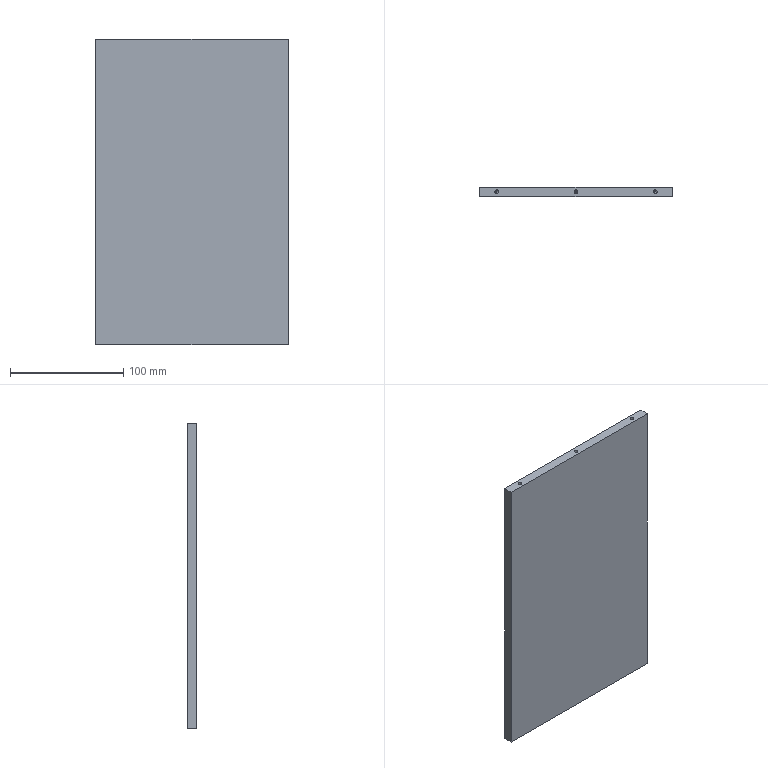Component | SolidWorks | LD101-02--Q1014-Q1-2-1 | 1 solid | 30 faces | box 170 x 8 x 270 mm | volume 366562 mm3 | cylinder 12 | cone 12 | plane 6 | commonest cylinder face diameters 3.3 x12 | material AL6061
build123d program:
from build123d import *

# Parameters (mm, degrees)
SKETCH1_W                  = 170
SKETCH1_H                  = 8
BOSS_EXTRUDE1_DEPTH        = 135
M4_TAPPED_HOLE1_AT_2_COUNT = 2
M4_TAPPED_HOLE1_AT_2_PITCH = 140
M4_TAPPED_HOLE1_AT_3_COUNT = 2
M4_TAPPED_HOLE1_AT_3_PITCH = 70


with BuildPart() as part:
    # Sketch1 → Boss-Extrude1 (new, symmetric)
    with BuildSketch(Plane.XY):
        Rectangle(SKETCH1_W, SKETCH1_H)
    extrude(amount=BOSS_EXTRUDE1_DEPTH, both=True)

    # Sketch2 → M4 Tapped Hole1 (revolve, cut)
    with BuildSketch(Plane(origin=(70, 0, -135), x_dir=(0, 1, 0), z_dir=(1, 0, 0))):
        Polygon((0, 0), (0, 13.091), (1.65, 12.1), (1.65, 0), align=None)
    m4_tapped_hole1 = revolve(axis=Axis((70, 0, -141.35), (0, 0, 1)), mode=Mode.SUBTRACT)

    # M4 Tapped Hole1 at 2: M4 Tapped Hole1 ×2
    with Locations(*[(-i * M4_TAPPED_HOLE1_AT_2_PITCH, 0, 0) for i in range(1, M4_TAPPED_HOLE1_AT_2_COUNT)]):
        add(m4_tapped_hole1, mode=Mode.SUBTRACT)

    # M4 Tapped Hole1 at 3: M4 Tapped Hole1 ×2
    with Locations(*[(-i * M4_TAPPED_HOLE1_AT_3_PITCH, 0, 0) for i in range(1, M4_TAPPED_HOLE1_AT_3_COUNT)]):
        add(m4_tapped_hole1, mode=Mode.SUBTRACT)

    # Mirror1: M4 Tapped Hole1 across plane
    add(m4_tapped_hole1.mirror(Plane.XY), mode=Mode.SUBTRACT)

    # Mirror1 copy 1 sketch → Mirror1 copy 1 (revolve, cut)
    with BuildSketch(Plane(origin=(-70, 0, 135), x_dir=(0, 1, 0), z_dir=(1, 0, 0))):
        Polygon((0, 0), (0, -13.091), (1.65, -12.1), (1.65, 0), align=None)
    revolve(axis=Axis((-70, 0, 141.35), (0, 0, 1)), mode=Mode.SUBTRACT)

    # Mirror1 copy 2 sketch → Mirror1 copy 2 (revolve, cut)
    with BuildSketch(Plane(origin=(0, 0, 135), x_dir=(0, 1, 0), z_dir=(1, 0, 0))):
        Polygon((0, 0), (0, -13.091), (1.65, -12.1), (1.65, 0), align=None)
    revolve(axis=Axis((0, 0, 141.35), (0, 0, 1)), mode=Mode.SUBTRACT)


solid = part.part

# Placed as in the assembly
solid = solid.moved(Location((244.21, -200.897, 146.257), (0, 0, 0)))
STEP:
#1=COLOUR_RGB('',0.7922,0.8196,0.9333);
#2=FILL_AREA_STYLE_COLOUR('',#1);
#3=FILL_AREA_STYLE('',(#2));
#4=SURFACE_STYLE_FILL_AREA(#3);
#5=SURFACE_SIDE_STYLE('',(#4));
#6=SURFACE_STYLE_USAGE(.BOTH.,#5);
#7=PRESENTATION_STYLE_ASSIGNMENT((#6));
#8=CARTESIAN_POINT('',(12.306,-7.909,10.597));
#9=VERTEX_POINT('',#8);
#10=CARTESIAN_POINT('',(12.435,-7.909,10.597));
#11=VERTEX_POINT('',#10);
#12=CARTESIAN_POINT('',(12.37,-7.909,10.597));
#13=DIRECTION('',(0.,0.,1.));
#14=DIRECTION('',(1.,0.,0.));
#15=AXIS2_PLACEMENT_3D('',#12,#13,#14);
#16=CIRCLE('',#15,0.06496);
#17=EDGE_CURVE('',#9,#11,#16,.T.);
#18=ORIENTED_EDGE('',*,*,#17,.F.);
#19=CARTESIAN_POINT('',(12.306,-7.909,11.073));
#20=VERTEX_POINT('',#19);
#21=CARTESIAN_POINT('',(12.306,-7.909,11.073));
#22=DIRECTION('',(0.,0.,1.));
#23=VECTOR('',#22,39.37);
#24=LINE('',#21,#23);
#25=EDGE_CURVE('',#9,#20,#24,.T.);
#26=ORIENTED_EDGE('',*,*,#25,.T.);
#27=CARTESIAN_POINT('',(12.435,-7.909,11.073));
#28=VERTEX_POINT('',#27);
#29=CARTESIAN_POINT('',(12.37,-7.909,11.073));
#30=DIRECTION('',(0.,0.,1.));
#31=DIRECTION('',(1.,0.,0.));
#32=AXIS2_PLACEMENT_3D('',#29,#30,#31);
#33=CIRCLE('',#32,0.06496);
#34=EDGE_CURVE('',#20,#28,#33,.T.);
#35=ORIENTED_EDGE('',*,*,#34,.T.);
#36=CARTESIAN_POINT('',(12.435,-7.909,11.073));
#37=DIRECTION('',(0.,0.,1.));
#38=VECTOR('',#37,39.37);
#39=LINE('',#36,#38);
#40=EDGE_CURVE('',#11,#28,#39,.T.);
#41=ORIENTED_EDGE('',*,*,#40,.F.);
#42=EDGE_LOOP('',(#18,#26,#35,#41));
#43=FACE_OUTER_BOUND('',#42,.T.);
#44=CARTESIAN_POINT('',(12.37,-7.909,11.073));
#45=DIRECTION('',(0.,0.,1.));
#46=DIRECTION('',(1.,0.,0.));
#47=AXIS2_PLACEMENT_3D('',#44,#45,#46);
#48=CYLINDRICAL_SURFACE('',#47,0.06496);
#49=ADVANCED_FACE('',(#43),#48,.F.);
#50=CARTESIAN_POINT('',(12.37,-7.909,10.558));
#51=VERTEX_POINT('',#50);
#52=CARTESIAN_POINT('',(12.435,-7.909,10.597));
#53=DIRECTION('',(0.8572,0.,0.515));
#54=VECTOR('',#53,39.37);
#55=LINE('',#52,#54);
#56=EDGE_CURVE('',#51,#11,#55,.T.);
#57=ORIENTED_EDGE('',*,*,#56,.F.);
#58=CARTESIAN_POINT('',(12.306,-7.909,10.597));
#59=DIRECTION('',(-0.8572,0.,0.515));
#60=VECTOR('',#59,39.37);
#61=LINE('',#58,#60);
#62=EDGE_CURVE('',#51,#9,#61,.T.);
#63=ORIENTED_EDGE('',*,*,#62,.T.);
#64=ORIENTED_EDGE('',*,*,#17,.T.);
#65=EDGE_LOOP('',(#57,#63,#64));
#66=FACE_OUTER_BOUND('',#65,.T.);
#67=CARTESIAN_POINT('',(12.37,-7.909,10.597));
#68=DIRECTION('',(0.,0.,1.));
#69=DIRECTION('',(1.,0.,0.));
#70=AXIS2_PLACEMENT_3D('',#67,#68,#69);
#71=CONICAL_SURFACE('',#70,0.06496,1.03);
#72=ADVANCED_FACE('',(#66),#71,.F.);
#73=CARTESIAN_POINT('',(6.794,-7.909,10.597));
#74=VERTEX_POINT('',#73);
#75=CARTESIAN_POINT('',(6.924,-7.909,10.597));
#76=VERTEX_POINT('',#75);
#77=CARTESIAN_POINT('',(6.859,-7.909,10.597));
#78=DIRECTION('',(0.,0.,1.));
#79=DIRECTION('',(1.,0.,0.));
#80=AXIS2_PLACEMENT_3D('',#77,#78,#79);
#81=CIRCLE('',#80,0.06496);
#82=EDGE_CURVE('',#74,#76,#81,.T.);
#83=ORIENTED_EDGE('',*,*,#82,.F.);
#84=CARTESIAN_POINT('',(6.794,-7.909,11.073));
#85=VERTEX_POINT('',#84);
#86=CARTESIAN_POINT('',(6.794,-7.909,11.073));
#87=DIRECTION('',(0.,0.,1.));
#88=VECTOR('',#87,39.37);
#89=LINE('',#86,#88);
#90=EDGE_CURVE('',#74,#85,#89,.T.);
#91=ORIENTED_EDGE('',*,*,#90,.T.);
#92=CARTESIAN_POINT('',(6.924,-7.909,11.073));
#93=VERTEX_POINT('',#92);
#94=CARTESIAN_POINT('',(6.859,-7.909,11.073));
#95=DIRECTION('',(0.,0.,1.));
#96=DIRECTION('',(1.,0.,0.));
#97=AXIS2_PLACEMENT_3D('',#94,#95,#96);
#98=CIRCLE('',#97,0.06496);
#99=EDGE_CURVE('',#85,#93,#98,.T.);
#100=ORIENTED_EDGE('',*,*,#99,.T.);
#101=CARTESIAN_POINT('',(6.924,-7.909,11.073));
#102=DIRECTION('',(0.,0.,1.));
#103=VECTOR('',#102,39.37);
#104=LINE('',#101,#103);
#105=EDGE_CURVE('',#76,#93,#104,.T.);
#106=ORIENTED_EDGE('',*,*,#105,.F.);
#107=EDGE_LOOP('',(#83,#91,#100,#106));
#108=FACE_OUTER_BOUND('',#107,.T.);
#109=CARTESIAN_POINT('',(6.859,-7.909,11.073));
#110=DIRECTION('',(0.,0.,1.));
#111=DIRECTION('',(1.,0.,0.));
#112=AXIS2_PLACEMENT_3D('',#109,#110,#111);
#113=CYLINDRICAL_SURFACE('',#112,0.06496);
#114=ADVANCED_FACE('',(#108),#113,.F.);
#115=CARTESIAN_POINT('',(6.859,-7.909,10.558));
#116=VERTEX_POINT('',#115);
#117=CARTESIAN_POINT('',(6.924,-7.909,10.597));
#118=DIRECTION('',(0.8572,0.,0.515));
#119=VECTOR('',#118,39.37);
#120=LINE('',#117,#119);
#121=EDGE_CURVE('',#116,#76,#120,.T.);
#122=ORIENTED_EDGE('',*,*,#121,.F.);
#123=CARTESIAN_POINT('',(6.794,-7.909,10.597));
#124=DIRECTION('',(-0.8572,0.,0.515));
#125=VECTOR('',#124,39.37);
#126=LINE('',#123,#125);
#127=EDGE_CURVE('',#116,#74,#126,.T.);
#128=ORIENTED_EDGE('',*,*,#127,.T.);
#129=ORIENTED_EDGE('',*,*,#82,.T.);
#130=EDGE_LOOP('',(#122,#128,#129));
#131=FACE_OUTER_BOUND('',#130,.T.);
#132=CARTESIAN_POINT('',(6.859,-7.909,10.597));
#133=DIRECTION('',(0.,0.,1.));
#134=DIRECTION('',(1.,0.,0.));
#135=AXIS2_PLACEMENT_3D('',#132,#133,#134);
#136=CONICAL_SURFACE('',#135,0.06496,1.03);
#137=ADVANCED_FACE('',(#131),#136,.F.);
#138=CARTESIAN_POINT('',(9.55,-7.909,10.597));
#139=VERTEX_POINT('',#138);
#140=CARTESIAN_POINT('',(9.68,-7.909,10.597));
#141=VERTEX_POINT('',#140);
#142=CARTESIAN_POINT('',(9.615,-7.909,10.597));
#143=DIRECTION('',(0.,0.,1.));
#144=DIRECTION('',(1.,0.,0.));
#145=AXIS2_PLACEMENT_3D('',#142,#143,#144);
#146=CIRCLE('',#145,0.06496);
#147=EDGE_CURVE('',#139,#141,#146,.T.);
#148=ORIENTED_EDGE('',*,*,#147,.F.);
#149=CARTESIAN_POINT('',(9.55,-7.909,11.073));
#150=VERTEX_POINT('',#149);
#151=CARTESIAN_POINT('',(9.55,-7.909,11.073));
#152=DIRECTION('',(0.,0.,1.));
#153=VECTOR('',#152,39.37);
#154=LINE('',#151,#153);
#155=EDGE_CURVE('',#139,#150,#154,.T.);
#156=ORIENTED_EDGE('',*,*,#155,.T.);
#157=CARTESIAN_POINT('',(9.68,-7.909,11.073));
#158=VERTEX_POINT('',#157);
#159=CARTESIAN_POINT('',(9.615,-7.909,11.073));
#160=DIRECTION('',(0.,0.,1.));
#161=DIRECTION('',(1.,0.,0.));
#162=AXIS2_PLACEMENT_3D('',#159,#160,#161);
#163=CIRCLE('',#162,0.06496);
#164=EDGE_CURVE('',#150,#158,#163,.T.);
#165=ORIENTED_EDGE('',*,*,#164,.T.);
#166=CARTESIAN_POINT('',(9.68,-7.909,11.073));
#167=DIRECTION('',(0.,0.,1.));
#168=VECTOR('',#167,39.37);
#169=LINE('',#166,#168);
#170=EDGE_CURVE('',#141,#158,#169,.T.);
#171=ORIENTED_EDGE('',*,*,#170,.F.);
#172=EDGE_LOOP('',(#148,#156,#165,#171));
#173=FACE_OUTER_BOUND('',#172,.T.);
#174=CARTESIAN_POINT('',(9.615,-7.909,11.073));
#175=DIRECTION('',(0.,0.,1.));
#176=DIRECTION('',(1.,0.,0.));
#177=AXIS2_PLACEMENT_3D('',#174,#175,#176);
#178=CYLINDRICAL_SURFACE('',#177,0.06496);
#179=ADVANCED_FACE('',(#173),#178,.F.);
#180=CARTESIAN_POINT('',(9.615,-7.909,10.558));
#181=VERTEX_POINT('',#180);
#182=CARTESIAN_POINT('',(9.68,-7.909,10.597));
#183=DIRECTION('',(0.8572,0.,0.515));
#184=VECTOR('',#183,39.37);
#185=LINE('',#182,#184);
#186=EDGE_CURVE('',#181,#141,#185,.T.);
#187=ORIENTED_EDGE('',*,*,#186,.F.);
#188=CARTESIAN_POINT('',(9.55,-7.909,10.597));
#189=DIRECTION('',(-0.8572,0.,0.515));
#190=VECTOR('',#189,39.37);
#191=LINE('',#188,#190);
#192=EDGE_CURVE('',#181,#139,#191,.T.);
#193=ORIENTED_EDGE('',*,*,#192,.T.);
#194=ORIENTED_EDGE('',*,*,#147,.T.);
#195=EDGE_LOOP('',(#187,#193,#194));
#196=FACE_OUTER_BOUND('',#195,.T.);
#197=CARTESIAN_POINT('',(9.615,-7.909,10.597));
#198=DIRECTION('',(0.,0.,1.));
#199=DIRECTION('',(1.,0.,0.));
#200=AXIS2_PLACEMENT_3D('',#197,#198,#199);
#201=CONICAL_SURFACE('',#200,0.06496,1.03);
#202=ADVANCED_FACE('',(#196),#201,.F.);
#203=CARTESIAN_POINT('',(12.435,-7.909,0.9196));
#204=VERTEX_POINT('',#203);
#205=CARTESIAN_POINT('',(12.306,-7.909,0.9196));
#206=VERTEX_POINT('',#205);
#207=CARTESIAN_POINT('',(12.37,-7.909,0.9196));
#208=DIRECTION('',(0.,0.,-1.));
#209=DIRECTION('',(-1.,0.,0.));
#210=AXIS2_PLACEMENT_3D('',#207,#208,#209);
#211=CIRCLE('',#210,0.06496);
#212=EDGE_CURVE('',#204,#206,#211,.T.);
#213=ORIENTED_EDGE('',*,*,#212,.F.);
#214=CARTESIAN_POINT('',(12.435,-7.909,0.4432));
#215=VERTEX_POINT('',#214);
#216=CARTESIAN_POINT('',(12.435,-7.909,0.4432));
#217=DIRECTION('',(0.,0.,-1.));
#218=VECTOR('',#217,39.37);
#219=LINE('',#216,#218);
#220=EDGE_CURVE('',#204,#215,#219,.T.);
#221=ORIENTED_EDGE('',*,*,#220,.T.);
#222=CARTESIAN_POINT('',(12.306,-7.909,0.4432));
#223=VERTEX_POINT('',#222);
#224=CARTESIAN_POINT('',(12.37,-7.909,0.4432));
#225=DIRECTION('',(0.,0.,-1.));
#226=DIRECTION('',(-1.,0.,0.));
#227=AXIS2_PLACEMENT_3D('',#224,#225,#226);
#228=CIRCLE('',#227,0.06496);
#229=EDGE_CURVE('',#215,#223,#228,.T.);
#230=ORIENTED_EDGE('',*,*,#229,.T.);
#231=CARTESIAN_POINT('',(12.306,-7.909,0.4432));
#232=DIRECTION('',(0.,0.,-1.));
#233=VECTOR('',#232,39.37);
#234=LINE('',#231,#233);
#235=EDGE_CURVE('',#206,#223,#234,.T.);
#236=ORIENTED_EDGE('',*,*,#235,.F.);
#237=EDGE_LOOP('',(#213,#221,#230,#236));
#238=FACE_OUTER_BOUND('',#237,.T.);
#239=CARTESIAN_POINT('',(12.37,-7.909,0.4432));
#240=DIRECTION('',(0.,0.,-1.));
#241=DIRECTION('',(-1.,0.,0.));
#242=AXIS2_PLACEMENT_3D('',#239,#240,#241);
#243=CYLINDRICAL_SURFACE('',#242,0.06496);
#244=ADVANCED_FACE('',(#238),#243,.F.);
#245=CARTESIAN_POINT('',(12.37,-7.909,0.9586));
#246=VERTEX_POINT('',#245);
#247=CARTESIAN_POINT('',(12.306,-7.909,0.9196));
#248=DIRECTION('',(-0.8572,0.,-0.515));
#249=VECTOR('',#248,39.37);
#250=LINE('',#247,#249);
#251=EDGE_CURVE('',#246,#206,#250,.T.);
#252=ORIENTED_EDGE('',*,*,#251,.F.);
#253=CARTESIAN_POINT('',(12.435,-7.909,0.9196));
#254=DIRECTION('',(0.8572,0.,-0.515));
#255=VECTOR('',#254,39.37);
#256=LINE('',#253,#255);
#257=EDGE_CURVE('',#246,#204,#256,.T.);
#258=ORIENTED_EDGE('',*,*,#257,.T.);
#259=ORIENTED_EDGE('',*,*,#212,.T.);
#260=EDGE_LOOP('',(#252,#258,#259));
#261=FACE_OUTER_BOUND('',#260,.T.);
#262=CARTESIAN_POINT('',(12.37,-7.909,0.9196));
#263=DIRECTION('',(0.,0.,-1.));
#264=DIRECTION('',(-1.,0.,0.));
#265=AXIS2_PLACEMENT_3D('',#262,#263,#264);
#266=CONICAL_SURFACE('',#265,0.06496,1.03);
#267=ADVANCED_FACE('',(#261),#266,.F.);
#268=CARTESIAN_POINT('',(6.924,-7.909,0.9196));
#269=VERTEX_POINT('',#268);
#270=CARTESIAN_POINT('',(6.794,-7.909,0.9196));
#271=VERTEX_POINT('',#270);
#272=CARTESIAN_POINT('',(6.859,-7.909,0.9196));
#273=DIRECTION('',(0.,0.,-1.));
#274=DIRECTION('',(-1.,0.,0.));
#275=AXIS2_PLACEMENT_3D('',#272,#273,#274);
#276=CIRCLE('',#275,0.06496);
#277=EDGE_CURVE('',#269,#271,#276,.T.);
#278=ORIENTED_EDGE('',*,*,#277,.F.);
#279=CARTESIAN_POINT('',(6.924,-7.909,0.4432));
#280=VERTEX_POINT('',#279);
#281=CARTESIAN_POINT('',(6.924,-7.909,0.4432));
#282=DIRECTION('',(0.,0.,-1.));
#283=VECTOR('',#282,39.37);
#284=LINE('',#281,#283);
#285=EDGE_CURVE('',#269,#280,#284,.T.);
#286=ORIENTED_EDGE('',*,*,#285,.T.);
#287=CARTESIAN_POINT('',(6.794,-7.909,0.4432));
#288=VERTEX_POINT('',#287);
#289=CARTESIAN_POINT('',(6.859,-7.909,0.4432));
#290=DIRECTION('',(0.,0.,-1.));
#291=DIRECTION('',(-1.,0.,0.));
#292=AXIS2_PLACEMENT_3D('',#289,#290,#291);
#293=CIRCLE('',#292,0.06496);
#294=EDGE_CURVE('',#280,#288,#293,.T.);
#295=ORIENTED_EDGE('',*,*,#294,.T.);
#296=CARTESIAN_POINT('',(6.794,-7.909,0.4432));
#297=DIRECTION('',(0.,0.,-1.));
#298=VECTOR('',#297,39.37);
#299=LINE('',#296,#298);
#300=EDGE_CURVE('',#271,#288,#299,.T.);
#301=ORIENTED_EDGE('',*,*,#300,.F.);
#302=EDGE_LOOP('',(#278,#286,#295,#301));
#303=FACE_OUTER_BOUND('',#302,.T.);
#304=CARTESIAN_POINT('',(6.859,-7.909,0.4432));
#305=DIRECTION('',(0.,0.,-1.));
#306=DIRECTION('',(-1.,0.,0.));
#307=AXIS2_PLACEMENT_3D('',#304,#305,#306);
#308=CYLINDRICAL_SURFACE('',#307,0.06496);
#309=ADVANCED_FACE('',(#303),#308,.F.);
#310=CARTESIAN_POINT('',(6.859,-7.909,0.9586));
#311=VERTEX_POINT('',#310);
#312=CARTESIAN_POINT('',(6.794,-7.909,0.9196));
#313=DIRECTION('',(-0.8572,0.,-0.515));
#314=VECTOR('',#313,39.37);
#315=LINE('',#312,#314);
#316=EDGE_CURVE('',#311,#271,#315,.T.);
#317=ORIENTED_EDGE('',*,*,#316,.F.);
#318=CARTESIAN_POINT('',(6.924,-7.909,0.9196));
#319=DIRECTION('',(0.8572,0.,-0.515));
#320=VECTOR('',#319,39.37);
#321=LINE('',#318,#320);
#322=EDGE_CURVE('',#311,#269,#321,.T.);
#323=ORIENTED_EDGE('',*,*,#322,.T.);
#324=ORIENTED_EDGE('',*,*,#277,.T.);
#325=EDGE_LOOP('',(#317,#323,#324));
#326=FACE_OUTER_BOUND('',#325,.T.);
#327=CARTESIAN_POINT('',(6.859,-7.909,0.9196));
#328=DIRECTION('',(0.,0.,-1.));
#329=DIRECTION('',(-1.,0.,0.));
#330=AXIS2_PLACEMENT_3D('',#327,#328,#329);
#331=CONICAL_SURFACE('',#330,0.06496,1.03);
#332=ADVANCED_FACE('',(#326),#331,.F.);
#333=CARTESIAN_POINT('',(9.68,-7.909,0.9196));
#334=VERTEX_POINT('',#333);
#335=CARTESIAN_POINT('',(9.55,-7.909,0.9196));
#336=VERTEX_POINT('',#335);
#337=CARTESIAN_POINT('',(9.615,-7.909,0.9196));
#338=DIRECTION('',(0.,0.,-1.));
#339=DIRECTION('',(-1.,0.,0.));
#340=AXIS2_PLACEMENT_3D('',#337,#338,#339);
#341=CIRCLE('',#340,0.06496);
#342=EDGE_CURVE('',#334,#336,#341,.T.);
#343=ORIENTED_EDGE('',*,*,#342,.F.);
#344=CARTESIAN_POINT('',(9.68,-7.909,0.4432));
#345=VERTEX_POINT('',#344);
#346=CARTESIAN_POINT('',(9.68,-7.909,0.4432));
#347=DIRECTION('',(0.,0.,-1.));
#348=VECTOR('',#347,39.37);
#349=LINE('',#346,#348);
#350=EDGE_CURVE('',#334,#345,#349,.T.);
#351=ORIENTED_EDGE('',*,*,#350,.T.);
#352=CARTESIAN_POINT('',(9.55,-7.909,0.4432));
#353=VERTEX_POINT('',#352);
#354=CARTESIAN_POINT('',(9.615,-7.909,0.4432));
#355=DIRECTION('',(0.,0.,-1.));
#356=DIRECTION('',(-1.,0.,0.));
#357=AXIS2_PLACEMENT_3D('',#354,#355,#356);
#358=CIRCLE('',#357,0.06496);
#359=EDGE_CURVE('',#345,#353,#358,.T.);
#360=ORIENTED_EDGE('',*,*,#359,.T.);
#361=CARTESIAN_POINT('',(9.55,-7.909,0.4432));
#362=DIRECTION('',(0.,0.,-1.));
#363=VECTOR('',#362,39.37);
#364=LINE('',#361,#363);
#365=EDGE_CURVE('',#336,#353,#364,.T.);
#366=ORIENTED_EDGE('',*,*,#365,.F.);
#367=EDGE_LOOP('',(#343,#351,#360,#366));
#368=FACE_OUTER_BOUND('',#367,.T.);
#369=CARTESIAN_POINT('',(9.615,-7.909,0.4432));
#370=DIRECTION('',(0.,0.,-1.));
#371=DIRECTION('',(-1.,0.,0.));
#372=AXIS2_PLACEMENT_3D('',#369,#370,#371);
#373=CYLINDRICAL_SURFACE('',#372,0.06496);
#374=ADVANCED_FACE('',(#368),#373,.F.);
#375=CARTESIAN_POINT('',(9.615,-7.909,0.9586));
#376=VERTEX_POINT('',#375);
#377=CARTESIAN_POINT('',(9.55,-7.909,0.9196));
#378=DIRECTION('',(-0.8572,0.,-0.515));
#379=VECTOR('',#378,39.37);
#380=LINE('',#377,#379);
#381=EDGE_CURVE('',#376,#336,#380,.T.);
#382=ORIENTED_EDGE('',*,*,#381,.F.);
#383=CARTESIAN_POINT('',(9.68,-7.909,0.9196));
#384=DIRECTION('',(0.8572,0.,-0.515));
#385=VECTOR('',#384,39.37);
#386=LINE('',#383,#385);
#387=EDGE_CURVE('',#376,#334,#386,.T.);
#388=ORIENTED_EDGE('',*,*,#387,.T.);
#389=ORIENTED_EDGE('',*,*,#342,.T.);
#390=EDGE_LOOP('',(#382,#388,#389));
#391=FACE_OUTER_BOUND('',#390,.T.);
#392=CARTESIAN_POINT('',(9.615,-7.909,0.9196));
#393=DIRECTION('',(0.,0.,-1.));
#394=DIRECTION('',(-1.,0.,0.));
#395=AXIS2_PLACEMENT_3D('',#392,#393,#394);
#396=CONICAL_SURFACE('',#395,0.06496,1.03);
#397=ADVANCED_FACE('',(#391),#396,.F.);
#398=CARTESIAN_POINT('',(12.961,-8.067,0.4432));
#399=VERTEX_POINT('',#398);
#400=CARTESIAN_POINT('',(12.961,-7.752,0.4432));
#401=VERTEX_POINT('',#400);
#402=CARTESIAN_POINT('',(12.961,-8.067,0.4432));
#403=DIRECTION('',(0.,1.,0.));
#404=VECTOR('',#403,39.37);
#405=LINE('',#402,#404);
#406=EDGE_CURVE('',#399,#401,#405,.T.);
#407=ORIENTED_EDGE('',*,*,#406,.T.);
#408=CARTESIAN_POINT('',(12.961,-7.752,11.073));
#409=VERTEX_POINT('',#408);
#410=CARTESIAN_POINT('',(12.961,-7.752,11.073));
#411=DIRECTION('',(0.,0.,-1.));
#412=VECTOR('',#411,39.37);
#413=LINE('',#410,#412);
#414=EDGE_CURVE('',#409,#401,#413,.T.);
#415=ORIENTED_EDGE('',*,*,#414,.F.);
#416=CARTESIAN_POINT('',(12.961,-8.067,11.073));
#417=VERTEX_POINT('',#416);
#418=CARTESIAN_POINT('',(12.961,-8.067,11.073));
#419=DIRECTION('',(0.,1.,0.));
#420=VECTOR('',#419,39.37);
#421=LINE('',#418,#420);
#422=EDGE_CURVE('',#417,#409,#421,.T.);
#423=ORIENTED_EDGE('',*,*,#422,.F.);
#424=CARTESIAN_POINT('',(12.961,-8.067,11.073));
#425=DIRECTION('',(0.,0.,-1.));
#426=VECTOR('',#425,39.37);
#427=LINE('',#424,#426);
#428=EDGE_CURVE('',#417,#399,#427,.T.);
#429=ORIENTED_EDGE('',*,*,#428,.T.);
#430=EDGE_LOOP('',(#407,#415,#423,#429));
#431=FACE_OUTER_BOUND('',#430,.T.);
#432=CARTESIAN_POINT('',(12.961,-8.067,11.073));
#433=DIRECTION('',(-1.,0.,0.));
#434=DIRECTION('',(0.,0.,1.));
#435=AXIS2_PLACEMENT_3D('',#432,#433,#434);
#436=PLANE('',#435);
#437=ADVANCED_FACE('',(#431),#436,.F.);
#438=CARTESIAN_POINT('',(6.268,-7.752,0.4432));
#439=VERTEX_POINT('',#438);
#440=CARTESIAN_POINT('',(6.268,-7.752,0.4432));
#441=DIRECTION('',(-1.,0.,0.));
#442=VECTOR('',#441,39.37);
#443=LINE('',#440,#442);
#444=EDGE_CURVE('',#401,#439,#443,.T.);
#445=ORIENTED_EDGE('',*,*,#444,.T.);
#446=CARTESIAN_POINT('',(6.268,-7.752,11.073));
#447=VERTEX_POINT('',#446);
#448=CARTESIAN_POINT('',(6.268,-7.752,11.073));
#449=DIRECTION('',(0.,0.,-1.));
#450=VECTOR('',#449,39.37);
#451=LINE('',#448,#450);
#452=EDGE_CURVE('',#447,#439,#451,.T.);
#453=ORIENTED_EDGE('',*,*,#452,.F.);
#454=CARTESIAN_POINT('',(6.268,-7.752,11.073));
#455=DIRECTION('',(-1.,0.,0.));
#456=VECTOR('',#455,39.37);
#457=LINE('',#454,#456);
#458=EDGE_CURVE('',#409,#447,#457,.T.);
#459=ORIENTED_EDGE('',*,*,#458,.F.);
#460=ORIENTED_EDGE('',*,*,#414,.T.);
#461=EDGE_LOOP('',(#445,#453,#459,#460));
#462=FACE_OUTER_BOUND('',#461,.T.);
#463=CARTESIAN_POINT('',(6.268,-7.752,11.073));
#464=DIRECTION('',(0.,-1.,0.));
#465=DIRECTION('',(0.,0.,-1.));
#466=AXIS2_PLACEMENT_3D('',#463,#464,#465);
#467=PLANE('',#466);
#468=ADVANCED_FACE('',(#462),#467,.F.);
#469=CARTESIAN_POINT('',(6.268,-8.067,0.4432));
#470=VERTEX_POINT('',#469);
#471=CARTESIAN_POINT('',(6.268,-8.067,0.4432));
#472=DIRECTION('',(0.,-1.,0.));
#473=VECTOR('',#472,39.37);
#474=LINE('',#471,#473);
#475=EDGE_CURVE('',#439,#470,#474,.T.);
#476=ORIENTED_EDGE('',*,*,#475,.T.);
#477=CARTESIAN_POINT('',(6.268,-8.067,11.073));
#478=VERTEX_POINT('',#477);
#479=CARTESIAN_POINT('',(6.268,-8.067,11.073));
#480=DIRECTION('',(0.,0.,-1.));
#481=VECTOR('',#480,39.37);
#482=LINE('',#479,#481);
#483=EDGE_CURVE('',#478,#470,#482,.T.);
#484=ORIENTED_EDGE('',*,*,#483,.F.);
#485=CARTESIAN_POINT('',(6.268,-8.067,11.073));
#486=DIRECTION('',(0.,-1.,0.));
#487=VECTOR('',#486,39.37);
#488=LINE('',#485,#487);
#489=EDGE_CURVE('',#447,#478,#488,.T.);
#490=ORIENTED_EDGE('',*,*,#489,.F.);
#491=ORIENTED_EDGE('',*,*,#452,.T.);
#492=EDGE_LOOP('',(#476,#484,#490,#491));
#493=FACE_OUTER_BOUND('',#492,.T.);
#494=CARTESIAN_POINT('',(6.268,-8.067,11.073));
#495=DIRECTION('',(1.,0.,0.));
#496=DIRECTION('',(0.,0.,-1.));
#497=AXIS2_PLACEMENT_3D('',#494,#495,#496);
#498=PLANE('',#497);
#499=ADVANCED_FACE('',(#493),#498,.F.);
#500=CARTESIAN_POINT('',(6.268,-8.067,0.4432));
#501=DIRECTION('',(1.,0.,0.));
#502=VECTOR('',#501,39.37);
#503=LINE('',#500,#502);
#504=EDGE_CURVE('',#470,#399,#503,.T.);
#505=ORIENTED_EDGE('',*,*,#504,.T.);
#506=ORIENTED_EDGE('',*,*,#428,.F.);
#507=CARTESIAN_POINT('',(6.268,-8.067,11.073));
#508=DIRECTION('',(1.,0.,0.));
#509=VECTOR('',#508,39.37);
#510=LINE('',#507,#509);
#511=EDGE_CURVE('',#478,#417,#510,.T.);
#512=ORIENTED_EDGE('',*,*,#511,.F.);
#513=ORIENTED_EDGE('',*,*,#483,.T.);
#514=EDGE_LOOP('',(#505,#506,#512,#513));
#515=FACE_OUTER_BOUND('',#514,.T.);
#516=CARTESIAN_POINT('',(6.268,-8.067,11.073));
#517=DIRECTION('',(0.,1.,0.));
#518=DIRECTION('',(0.,0.,1.));
#519=AXIS2_PLACEMENT_3D('',#516,#517,#518);
#520=PLANE('',#519);
#521=ADVANCED_FACE('',(#515),#520,.F.);
#522=CARTESIAN_POINT('',(12.37,-7.909,11.073));
#523=DIRECTION('',(0.,0.,1.));
#524=DIRECTION('',(1.,0.,0.));
#525=AXIS2_PLACEMENT_3D('',#522,#523,#524);
#526=CIRCLE('',#525,0.06496);
#527=EDGE_CURVE('',#28,#20,#526,.T.);
#528=ORIENTED_EDGE('',*,*,#527,.F.);
#529=ORIENTED_EDGE('',*,*,#34,.F.);
#530=EDGE_LOOP('',(#528,#529));
#531=FACE_BOUND('',#530,.T.);
#532=CARTESIAN_POINT('',(6.859,-7.909,11.073));
#533=DIRECTION('',(0.,0.,1.));
#534=DIRECTION('',(1.,0.,0.));
#535=AXIS2_PLACEMENT_3D('',#532,#533,#534);
#536=CIRCLE('',#535,0.06496);
#537=EDGE_CURVE('',#93,#85,#536,.T.);
#538=ORIENTED_EDGE('',*,*,#537,.F.);
#539=ORIENTED_EDGE('',*,*,#99,.F.);
#540=EDGE_LOOP('',(#538,#539));
#541=FACE_BOUND('',#540,.T.);
#542=CARTESIAN_POINT('',(9.615,-7.909,11.073));
#543=DIRECTION('',(0.,0.,1.));
#544=DIRECTION('',(1.,0.,0.));
#545=AXIS2_PLACEMENT_3D('',#542,#543,#544);
#546=CIRCLE('',#545,0.06496);
#547=EDGE_CURVE('',#158,#150,#546,.T.);
#548=ORIENTED_EDGE('',*,*,#547,.F.);
#549=ORIENTED_EDGE('',*,*,#164,.F.);
#550=EDGE_LOOP('',(#548,#549));
#551=FACE_BOUND('',#550,.T.);
#552=ORIENTED_EDGE('',*,*,#422,.T.);
#553=ORIENTED_EDGE('',*,*,#458,.T.);
#554=ORIENTED_EDGE('',*,*,#489,.T.);
#555=ORIENTED_EDGE('',*,*,#511,.T.);
#556=EDGE_LOOP('',(#552,#553,#554,#555));
#557=FACE_OUTER_BOUND('',#556,.T.);
#558=CARTESIAN_POINT('',(9.615,-7.909,11.073));
#559=DIRECTION('',(0.,0.,-1.));
#560=DIRECTION('',(-1.,0.,0.));
#561=AXIS2_PLACEMENT_3D('',#558,#559,#560);
#562=PLANE('',#561);
#563=ADVANCED_FACE('',(#531,#541,#551,#557),#562,.F.);
#564=CARTESIAN_POINT('',(12.37,-7.909,0.4432));
#565=DIRECTION('',(0.,0.,-1.));
#566=DIRECTION('',(-1.,0.,0.));
#567=AXIS2_PLACEMENT_3D('',#564,#565,#566);
#568=CIRCLE('',#567,0.06496);
#569=EDGE_CURVE('',#223,#215,#568,.T.);
#570=ORIENTED_EDGE('',*,*,#569,.F.);
#571=ORIENTED_EDGE('',*,*,#229,.F.);
#572=EDGE_LOOP('',(#570,#571));
#573=FACE_BOUND('',#572,.T.);
#574=CARTESIAN_POINT('',(6.859,-7.909,0.4432));
#575=DIRECTION('',(0.,0.,-1.));
#576=DIRECTION('',(-1.,0.,0.));
#577=AXIS2_PLACEMENT_3D('',#574,#575,#576);
#578=CIRCLE('',#577,0.06496);
#579=EDGE_CURVE('',#288,#280,#578,.T.);
#580=ORIENTED_EDGE('',*,*,#579,.F.);
#581=ORIENTED_EDGE('',*,*,#294,.F.);
#582=EDGE_LOOP('',(#580,#581));
#583=FACE_BOUND('',#582,.T.);
#584=CARTESIAN_POINT('',(9.615,-7.909,0.4432));
#585=DIRECTION('',(0.,0.,-1.));
#586=DIRECTION('',(-1.,0.,0.));
#587=AXIS2_PLACEMENT_3D('',#584,#585,#586);
#588=CIRCLE('',#587,0.06496);
#589=EDGE_CURVE('',#353,#345,#588,.T.);
#590=ORIENTED_EDGE('',*,*,#589,.F.);
#591=ORIENTED_EDGE('',*,*,#359,.F.);
#592=EDGE_LOOP('',(#590,#591));
#593=FACE_BOUND('',#592,.T.);
#594=ORIENTED_EDGE('',*,*,#406,.F.);
#595=ORIENTED_EDGE('',*,*,#504,.F.);
#596=ORIENTED_EDGE('',*,*,#475,.F.);
#597=ORIENTED_EDGE('',*,*,#444,.F.);
#598=EDGE_LOOP('',(#594,#595,#596,#597));
#599=FACE_OUTER_BOUND('',#598,.T.);
#600=CARTESIAN_POINT('',(9.615,-7.909,0.4432));
#601=DIRECTION('',(0.,0.,-1.));
#602=DIRECTION('',(-1.,0.,0.));
#603=AXIS2_PLACEMENT_3D('',#600,#601,#602);
#604=PLANE('',#603);
#605=ADVANCED_FACE('',(#573,#583,#593,#599),#604,.T.);
#606=ORIENTED_EDGE('',*,*,#387,.F.);
#607=ORIENTED_EDGE('',*,*,#381,.T.);
#608=CARTESIAN_POINT('',(9.615,-7.909,0.9196));
#609=DIRECTION('',(0.,0.,-1.));
#610=DIRECTION('',(-1.,0.,0.));
#611=AXIS2_PLACEMENT_3D('',#608,#609,#610);
#612=CIRCLE('',#611,0.06496);
#613=EDGE_CURVE('',#336,#334,#612,.T.);
#614=ORIENTED_EDGE('',*,*,#613,.T.);
#615=EDGE_LOOP('',(#606,#607,#614));
#616=FACE_OUTER_BOUND('',#615,.T.);
#617=CARTESIAN_POINT('',(9.615,-7.909,0.9196));
#618=DIRECTION('',(0.,0.,-1.));
#619=DIRECTION('',(-1.,0.,0.));
#620=AXIS2_PLACEMENT_3D('',#617,#618,#619);
#621=CONICAL_SURFACE('',#620,0.06496,1.03);
#622=ADVANCED_FACE('',(#616),#621,.F.);
#623=ORIENTED_EDGE('',*,*,#350,.F.);
#624=ORIENTED_EDGE('',*,*,#613,.F.);
#625=ORIENTED_EDGE('',*,*,#365,.T.);
#626=ORIENTED_EDGE('',*,*,#589,.T.);
#627=EDGE_LOOP('',(#623,#624,#625,#626));
#628=FACE_OUTER_BOUND('',#627,.T.);
#629=CARTESIAN_POINT('',(9.615,-7.909,0.4432));
#630=DIRECTION('',(0.,0.,-1.));
#631=DIRECTION('',(-1.,0.,0.));
#632=AXIS2_PLACEMENT_3D('',#629,#630,#631);
#633=CYLINDRICAL_SURFACE('',#632,0.06496);
#634=ADVANCED_FACE('',(#628),#633,.F.);
#635=ORIENTED_EDGE('',*,*,#322,.F.);
#636=ORIENTED_EDGE('',*,*,#316,.T.);
#637=CARTESIAN_POINT('',(6.859,-7.909,0.9196));
#638=DIRECTION('',(0.,0.,-1.));
#639=DIRECTION('',(-1.,0.,0.));
#640=AXIS2_PLACEMENT_3D('',#637,#638,#639);
#641=CIRCLE('',#640,0.06496);
#642=EDGE_CURVE('',#271,#269,#641,.T.);
#643=ORIENTED_EDGE('',*,*,#642,.T.);
#644=EDGE_LOOP('',(#635,#636,#643));
#645=FACE_OUTER_BOUND('',#644,.T.);
#646=CARTESIAN_POINT('',(6.859,-7.909,0.9196));
#647=DIRECTION('',(0.,0.,-1.));
#648=DIRECTION('',(-1.,0.,0.));
#649=AXIS2_PLACEMENT_3D('',#646,#647,#648);
#650=CONICAL_SURFACE('',#649,0.06496,1.03);
#651=ADVANCED_FACE('',(#645),#650,.F.);
#652=ORIENTED_EDGE('',*,*,#285,.F.);
#653=ORIENTED_EDGE('',*,*,#642,.F.);
#654=ORIENTED_EDGE('',*,*,#300,.T.);
#655=ORIENTED_EDGE('',*,*,#579,.T.);
#656=EDGE_LOOP('',(#652,#653,#654,#655));
#657=FACE_OUTER_BOUND('',#656,.T.);
#658=CARTESIAN_POINT('',(6.859,-7.909,0.4432));
#659=DIRECTION('',(0.,0.,-1.));
#660=DIRECTION('',(-1.,0.,0.));
#661=AXIS2_PLACEMENT_3D('',#658,#659,#660);
#662=CYLINDRICAL_SURFACE('',#661,0.06496);
#663=ADVANCED_FACE('',(#657),#662,.F.);
#664=ORIENTED_EDGE('',*,*,#257,.F.);
#665=ORIENTED_EDGE('',*,*,#251,.T.);
#666=CARTESIAN_POINT('',(12.37,-7.909,0.9196));
#667=DIRECTION('',(0.,0.,-1.));
#668=DIRECTION('',(-1.,0.,0.));
#669=AXIS2_PLACEMENT_3D('',#666,#667,#668);
#670=CIRCLE('',#669,0.06496);
#671=EDGE_CURVE('',#206,#204,#670,.T.);
#672=ORIENTED_EDGE('',*,*,#671,.T.);
#673=EDGE_LOOP('',(#664,#665,#672));
#674=FACE_OUTER_BOUND('',#673,.T.);
#675=CARTESIAN_POINT('',(12.37,-7.909,0.9196));
#676=DIRECTION('',(0.,0.,-1.));
#677=DIRECTION('',(-1.,0.,0.));
#678=AXIS2_PLACEMENT_3D('',#675,#676,#677);
#679=CONICAL_SURFACE('',#678,0.06496,1.03);
#680=ADVANCED_FACE('',(#674),#679,.F.);
#681=ORIENTED_EDGE('',*,*,#220,.F.);
#682=ORIENTED_EDGE('',*,*,#671,.F.);
#683=ORIENTED_EDGE('',*,*,#235,.T.);
#684=ORIENTED_EDGE('',*,*,#569,.T.);
#685=EDGE_LOOP('',(#681,#682,#683,#684));
#686=FACE_OUTER_BOUND('',#685,.T.);
#687=CARTESIAN_POINT('',(12.37,-7.909,0.4432));
#688=DIRECTION('',(0.,0.,-1.));
#689=DIRECTION('',(-1.,0.,0.));
#690=AXIS2_PLACEMENT_3D('',#687,#688,#689);
#691=CYLINDRICAL_SURFACE('',#690,0.06496);
#692=ADVANCED_FACE('',(#686),#691,.F.);
#693=ORIENTED_EDGE('',*,*,#192,.F.);
#694=ORIENTED_EDGE('',*,*,#186,.T.);
#695=CARTESIAN_POINT('',(9.615,-7.909,10.597));
#696=DIRECTION('',(0.,0.,1.));
#697=DIRECTION('',(1.,0.,0.));
#698=AXIS2_PLACEMENT_3D('',#695,#696,#697);
#699=CIRCLE('',#698,0.06496);
#700=EDGE_CURVE('',#141,#139,#699,.T.);
#701=ORIENTED_EDGE('',*,*,#700,.T.);
#702=EDGE_LOOP('',(#693,#694,#701));
#703=FACE_OUTER_BOUND('',#702,.T.);
#704=CARTESIAN_POINT('',(9.615,-7.909,10.597));
#705=DIRECTION('',(0.,0.,1.));
#706=DIRECTION('',(1.,0.,0.));
#707=AXIS2_PLACEMENT_3D('',#704,#705,#706);
#708=CONICAL_SURFACE('',#707,0.06496,1.03);
#709=ADVANCED_FACE('',(#703),#708,.F.);
#710=ORIENTED_EDGE('',*,*,#155,.F.);
#711=ORIENTED_EDGE('',*,*,#700,.F.);
#712=ORIENTED_EDGE('',*,*,#170,.T.);
#713=ORIENTED_EDGE('',*,*,#547,.T.);
#714=EDGE_LOOP('',(#710,#711,#712,#713));
#715=FACE_OUTER_BOUND('',#714,.T.);
#716=CARTESIAN_POINT('',(9.615,-7.909,11.073));
#717=DIRECTION('',(0.,0.,1.));
#718=DIRECTION('',(1.,0.,0.));
#719=AXIS2_PLACEMENT_3D('',#716,#717,#718);
#720=CYLINDRICAL_SURFACE('',#719,0.06496);
#721=ADVANCED_FACE('',(#715),#720,.F.);
#722=ORIENTED_EDGE('',*,*,#127,.F.);
#723=ORIENTED_EDGE('',*,*,#121,.T.);
#724=CARTESIAN_POINT('',(6.859,-7.909,10.597));
#725=DIRECTION('',(0.,0.,1.));
#726=DIRECTION('',(1.,0.,0.));
#727=AXIS2_PLACEMENT_3D('',#724,#725,#726);
#728=CIRCLE('',#727,0.06496);
#729=EDGE_CURVE('',#76,#74,#728,.T.);
#730=ORIENTED_EDGE('',*,*,#729,.T.);
#731=EDGE_LOOP('',(#722,#723,#730));
#732=FACE_OUTER_BOUND('',#731,.T.);
#733=CARTESIAN_POINT('',(6.859,-7.909,10.597));
#734=DIRECTION('',(0.,0.,1.));
#735=DIRECTION('',(1.,0.,0.));
#736=AXIS2_PLACEMENT_3D('',#733,#734,#735);
#737=CONICAL_SURFACE('',#736,0.06496,1.03);
#738=ADVANCED_FACE('',(#732),#737,.F.);
#739=ORIENTED_EDGE('',*,*,#90,.F.);
#740=ORIENTED_EDGE('',*,*,#729,.F.);
#741=ORIENTED_EDGE('',*,*,#105,.T.);
#742=ORIENTED_EDGE('',*,*,#537,.T.);
#743=EDGE_LOOP('',(#739,#740,#741,#742));
#744=FACE_OUTER_BOUND('',#743,.T.);
#745=CARTESIAN_POINT('',(6.859,-7.909,11.073));
#746=DIRECTION('',(0.,0.,1.));
#747=DIRECTION('',(1.,0.,0.));
#748=AXIS2_PLACEMENT_3D('',#745,#746,#747);
#749=CYLINDRICAL_SURFACE('',#748,0.06496);
#750=ADVANCED_FACE('',(#744),#749,.F.);
#751=ORIENTED_EDGE('',*,*,#62,.F.);
#752=ORIENTED_EDGE('',*,*,#56,.T.);
#753=CARTESIAN_POINT('',(12.37,-7.909,10.597));
#754=DIRECTION('',(0.,0.,1.));
#755=DIRECTION('',(1.,0.,0.));
#756=AXIS2_PLACEMENT_3D('',#753,#754,#755);
#757=CIRCLE('',#756,0.06496);
#758=EDGE_CURVE('',#11,#9,#757,.T.);
#759=ORIENTED_EDGE('',*,*,#758,.T.);
#760=EDGE_LOOP('',(#751,#752,#759));
#761=FACE_OUTER_BOUND('',#760,.T.);
#762=CARTESIAN_POINT('',(12.37,-7.909,10.597));
#763=DIRECTION('',(0.,0.,1.));
#764=DIRECTION('',(1.,0.,0.));
#765=AXIS2_PLACEMENT_3D('',#762,#763,#764);
#766=CONICAL_SURFACE('',#765,0.06496,1.03);
#767=ADVANCED_FACE('',(#761),#766,.F.);
#768=ORIENTED_EDGE('',*,*,#25,.F.);
#769=ORIENTED_EDGE('',*,*,#758,.F.);
#770=ORIENTED_EDGE('',*,*,#40,.T.);
#771=ORIENTED_EDGE('',*,*,#527,.T.);
#772=EDGE_LOOP('',(#768,#769,#770,#771));
#773=FACE_OUTER_BOUND('',#772,.T.);
#774=CARTESIAN_POINT('',(12.37,-7.909,11.073));
#775=DIRECTION('',(0.,0.,1.));
#776=DIRECTION('',(1.,0.,0.));
#777=AXIS2_PLACEMENT_3D('',#774,#775,#776);
#778=CYLINDRICAL_SURFACE('',#777,0.06496);
#779=ADVANCED_FACE('',(#773),#778,.F.);
#780=CLOSED_SHELL('',(#49,#72,#114,#137,#179,#202,#244,#267,#309,#332,#374,#397,#437,#468,#499,#521,#563,#605,#622,#634,#651,#663,#680,#692,#709,#721,#738,#750,#767,#779));
#781=MANIFOLD_SOLID_BREP('',#780);
#782=STYLED_ITEM('',(#7),#781);
#783=PRESENTATION_LAYER_ASSIGNMENT('','',(#782));
#784=(LENGTH_UNIT()NAMED_UNIT(*)SI_UNIT($,.METRE.));
#785=LENGTH_MEASURE_WITH_UNIT(LENGTH_MEASURE(0.0254),#784);
#786=DIMENSIONAL_EXPONENTS(1.,0.,0.,0.,0.,0.,0.);
#787=(CONVERSION_BASED_UNIT('',#785)LENGTH_UNIT()NAMED_UNIT(#786));
#788=UNCERTAINTY_MEASURE_WITH_UNIT(LENGTH_MEASURE(0.00001),#787,'','');
#789=(NAMED_UNIT(*)PLANE_ANGLE_UNIT()SI_UNIT($,.RADIAN.));
#790=(NAMED_UNIT(*)SI_UNIT($,.STERADIAN.)SOLID_ANGLE_UNIT());
#791=(GEOMETRIC_REPRESENTATION_CONTEXT(3)GLOBAL_UNCERTAINTY_ASSIGNED_CONTEXT((#788))GLOBAL_UNIT_ASSIGNED_CONTEXT((#787,#789,#790))REPRESENTATION_CONTEXT('',''));
#792=MECHANICAL_DESIGN_GEOMETRIC_PRESENTATION_REPRESENTATION('',(#782),#791);
#793=CARTESIAN_POINT('',(0.,0.,0.));
#794=DIRECTION('',(0.,0.,1.));
#795=DIRECTION('',(1.,0.,0.));
#796=AXIS2_PLACEMENT_3D('',#793,#794,#795);
#797=(LENGTH_UNIT()NAMED_UNIT(*)SI_UNIT($,.METRE.));
#798=LENGTH_MEASURE_WITH_UNIT(LENGTH_MEASURE(0.0254),#797);
#799=DIMENSIONAL_EXPONENTS(1.,0.,0.,0.,0.,0.,0.);
#800=(CONVERSION_BASED_UNIT('',#798)LENGTH_UNIT()NAMED_UNIT(#799));
#801=UNCERTAINTY_MEASURE_WITH_UNIT(LENGTH_MEASURE(0.00001),#800,'','');
#802=(NAMED_UNIT(*)PLANE_ANGLE_UNIT()SI_UNIT($,.RADIAN.));
#803=(NAMED_UNIT(*)SI_UNIT($,.STERADIAN.)SOLID_ANGLE_UNIT());
#804=(GEOMETRIC_REPRESENTATION_CONTEXT(3)GLOBAL_UNCERTAINTY_ASSIGNED_CONTEXT((#801))GLOBAL_UNIT_ASSIGNED_CONTEXT((#800,#802,#803))REPRESENTATION_CONTEXT('',''));
#805=ADVANCED_BREP_SHAPE_REPRESENTATION('',(#781,#796),#804);